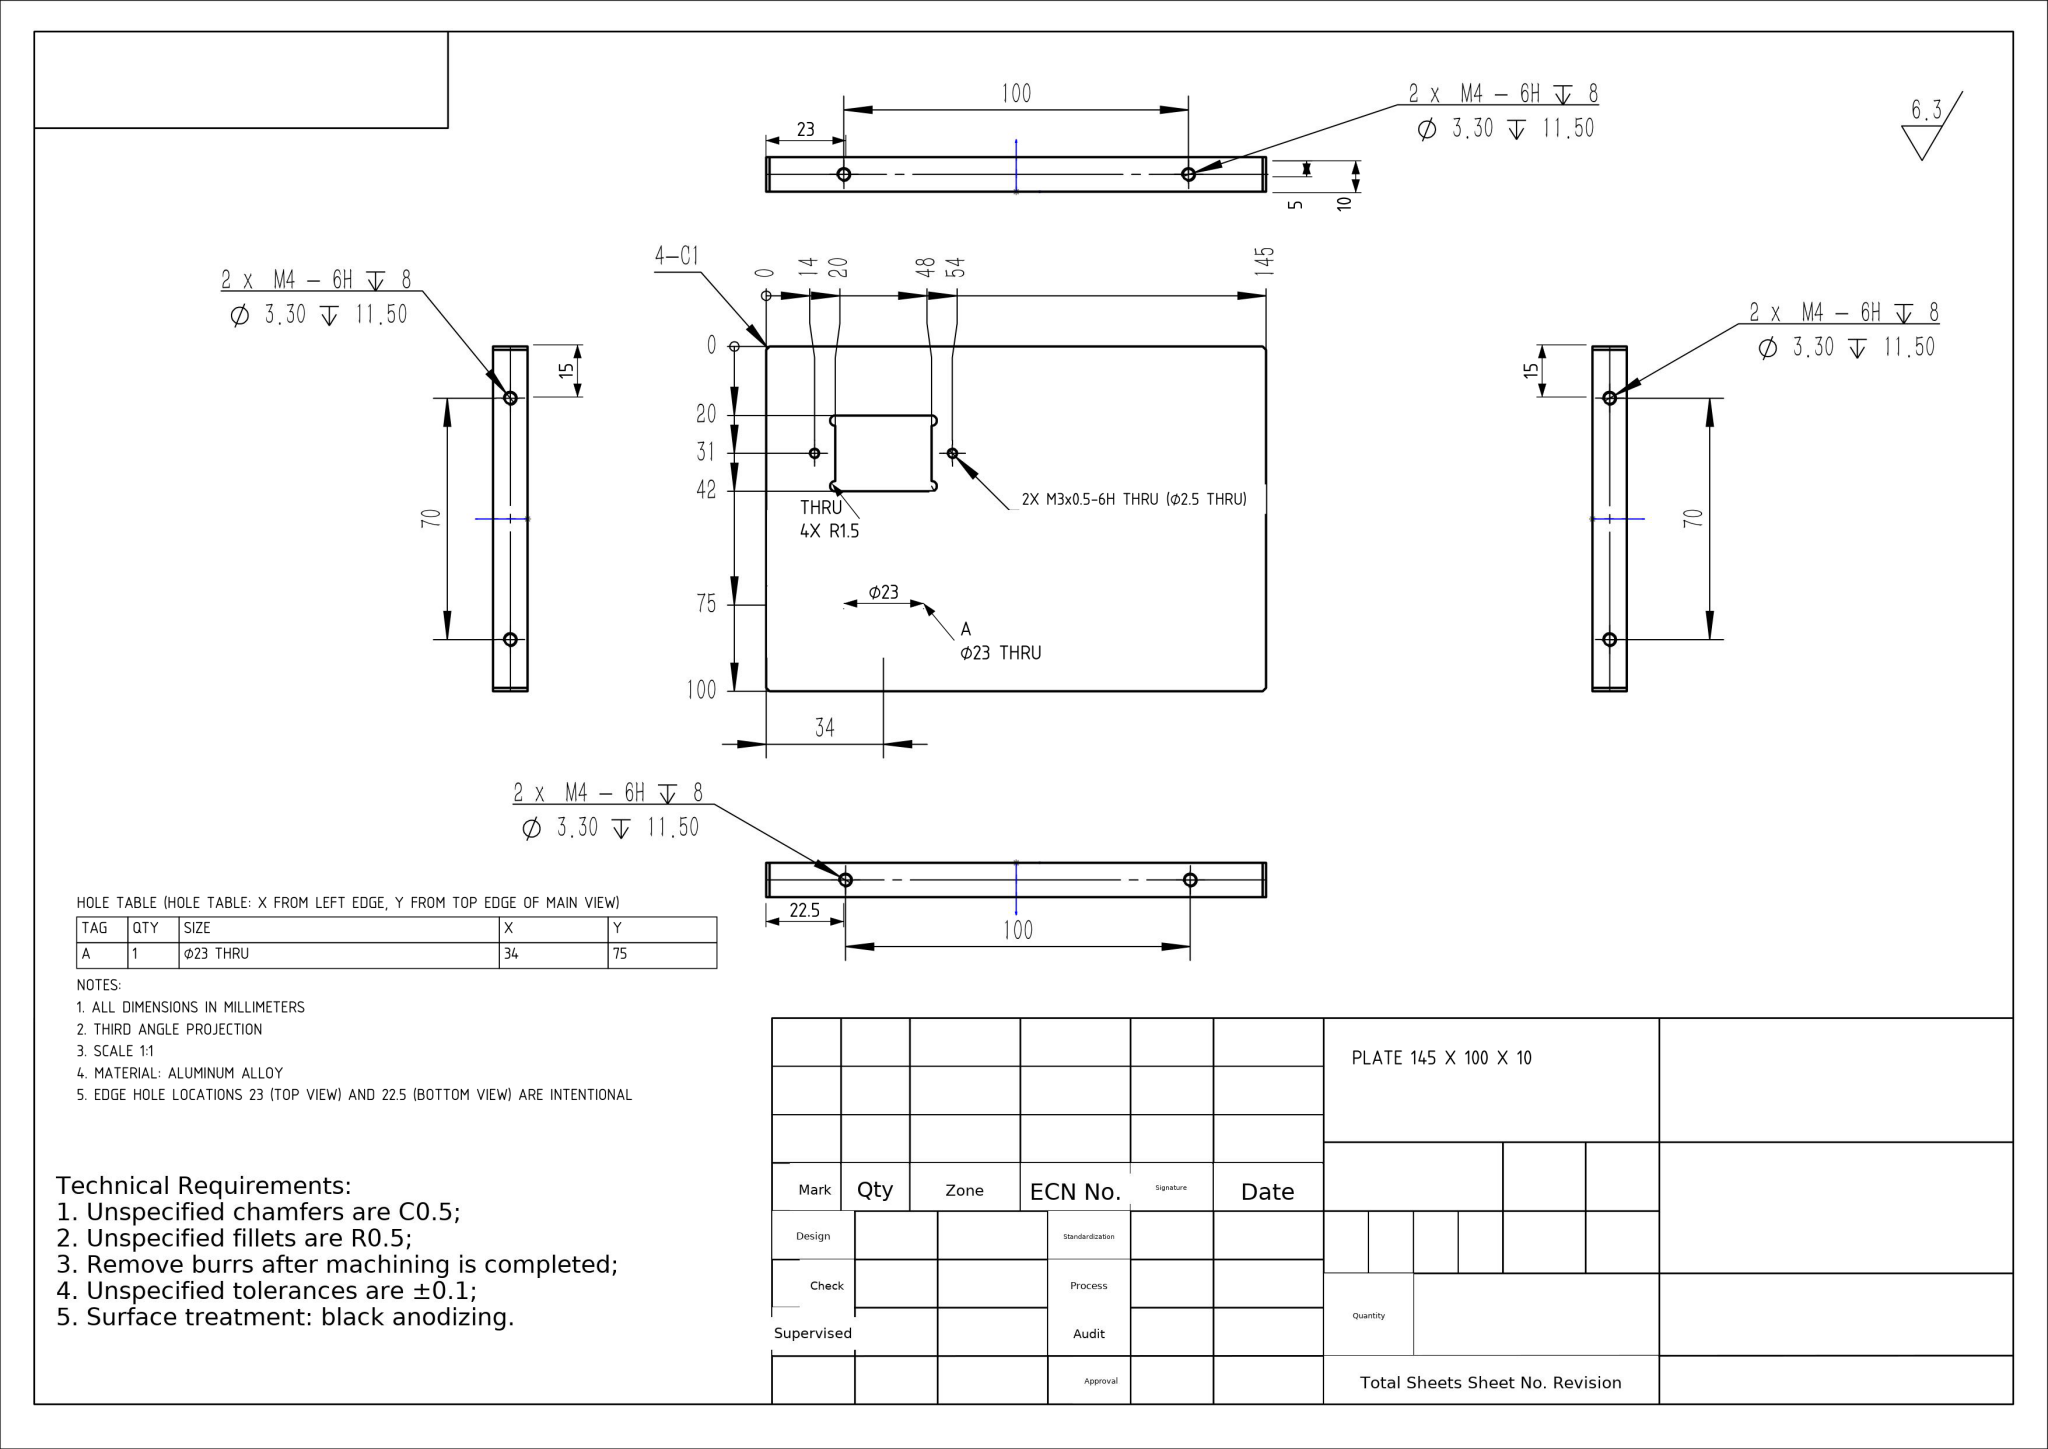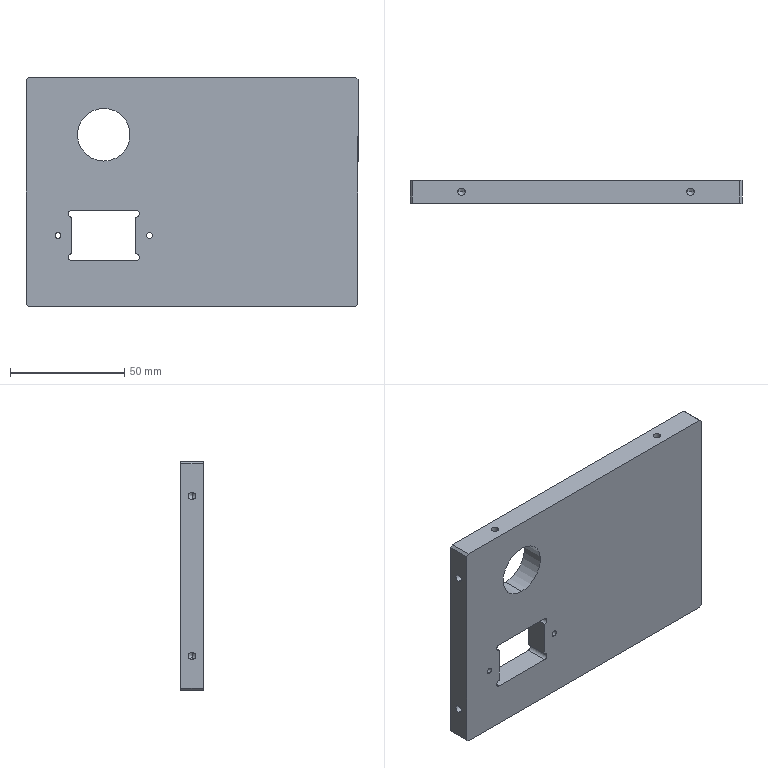Part | NX | mm | 1 solid | 56 faces | box 145 x 10 x 100 mm | volume 133616 mm3 | cylinder 26 | cone 16 | plane 14 | commonest cylinder face diameters 3.3 x16 2.5 x4 3 x4 23 x2